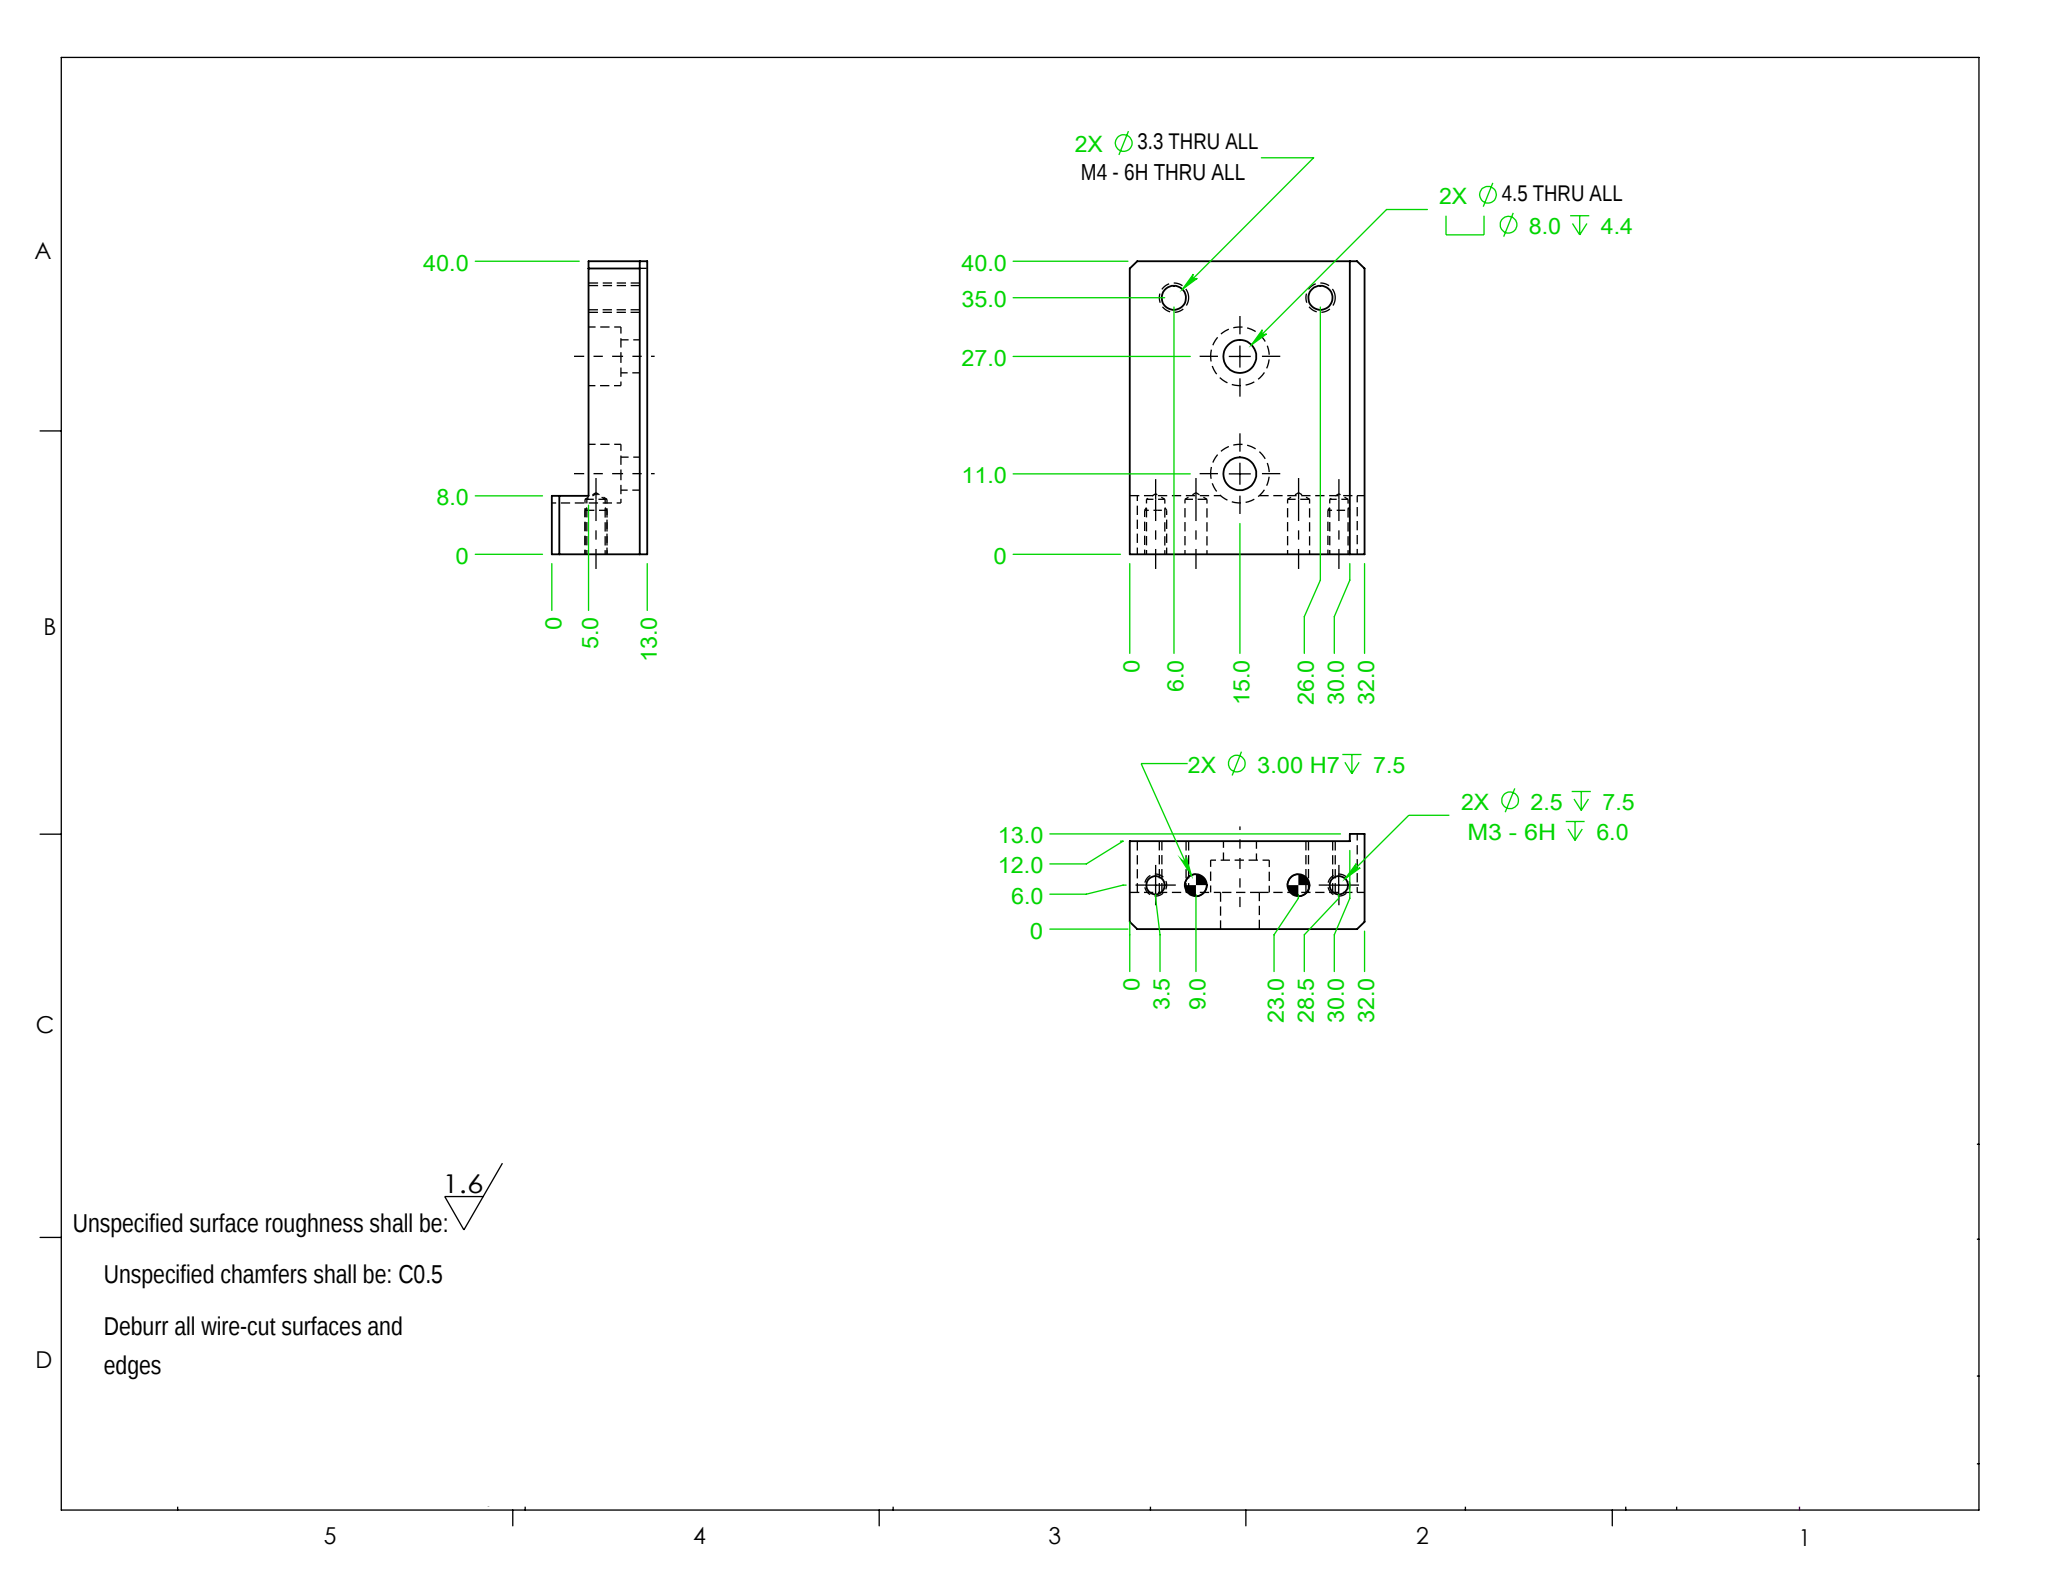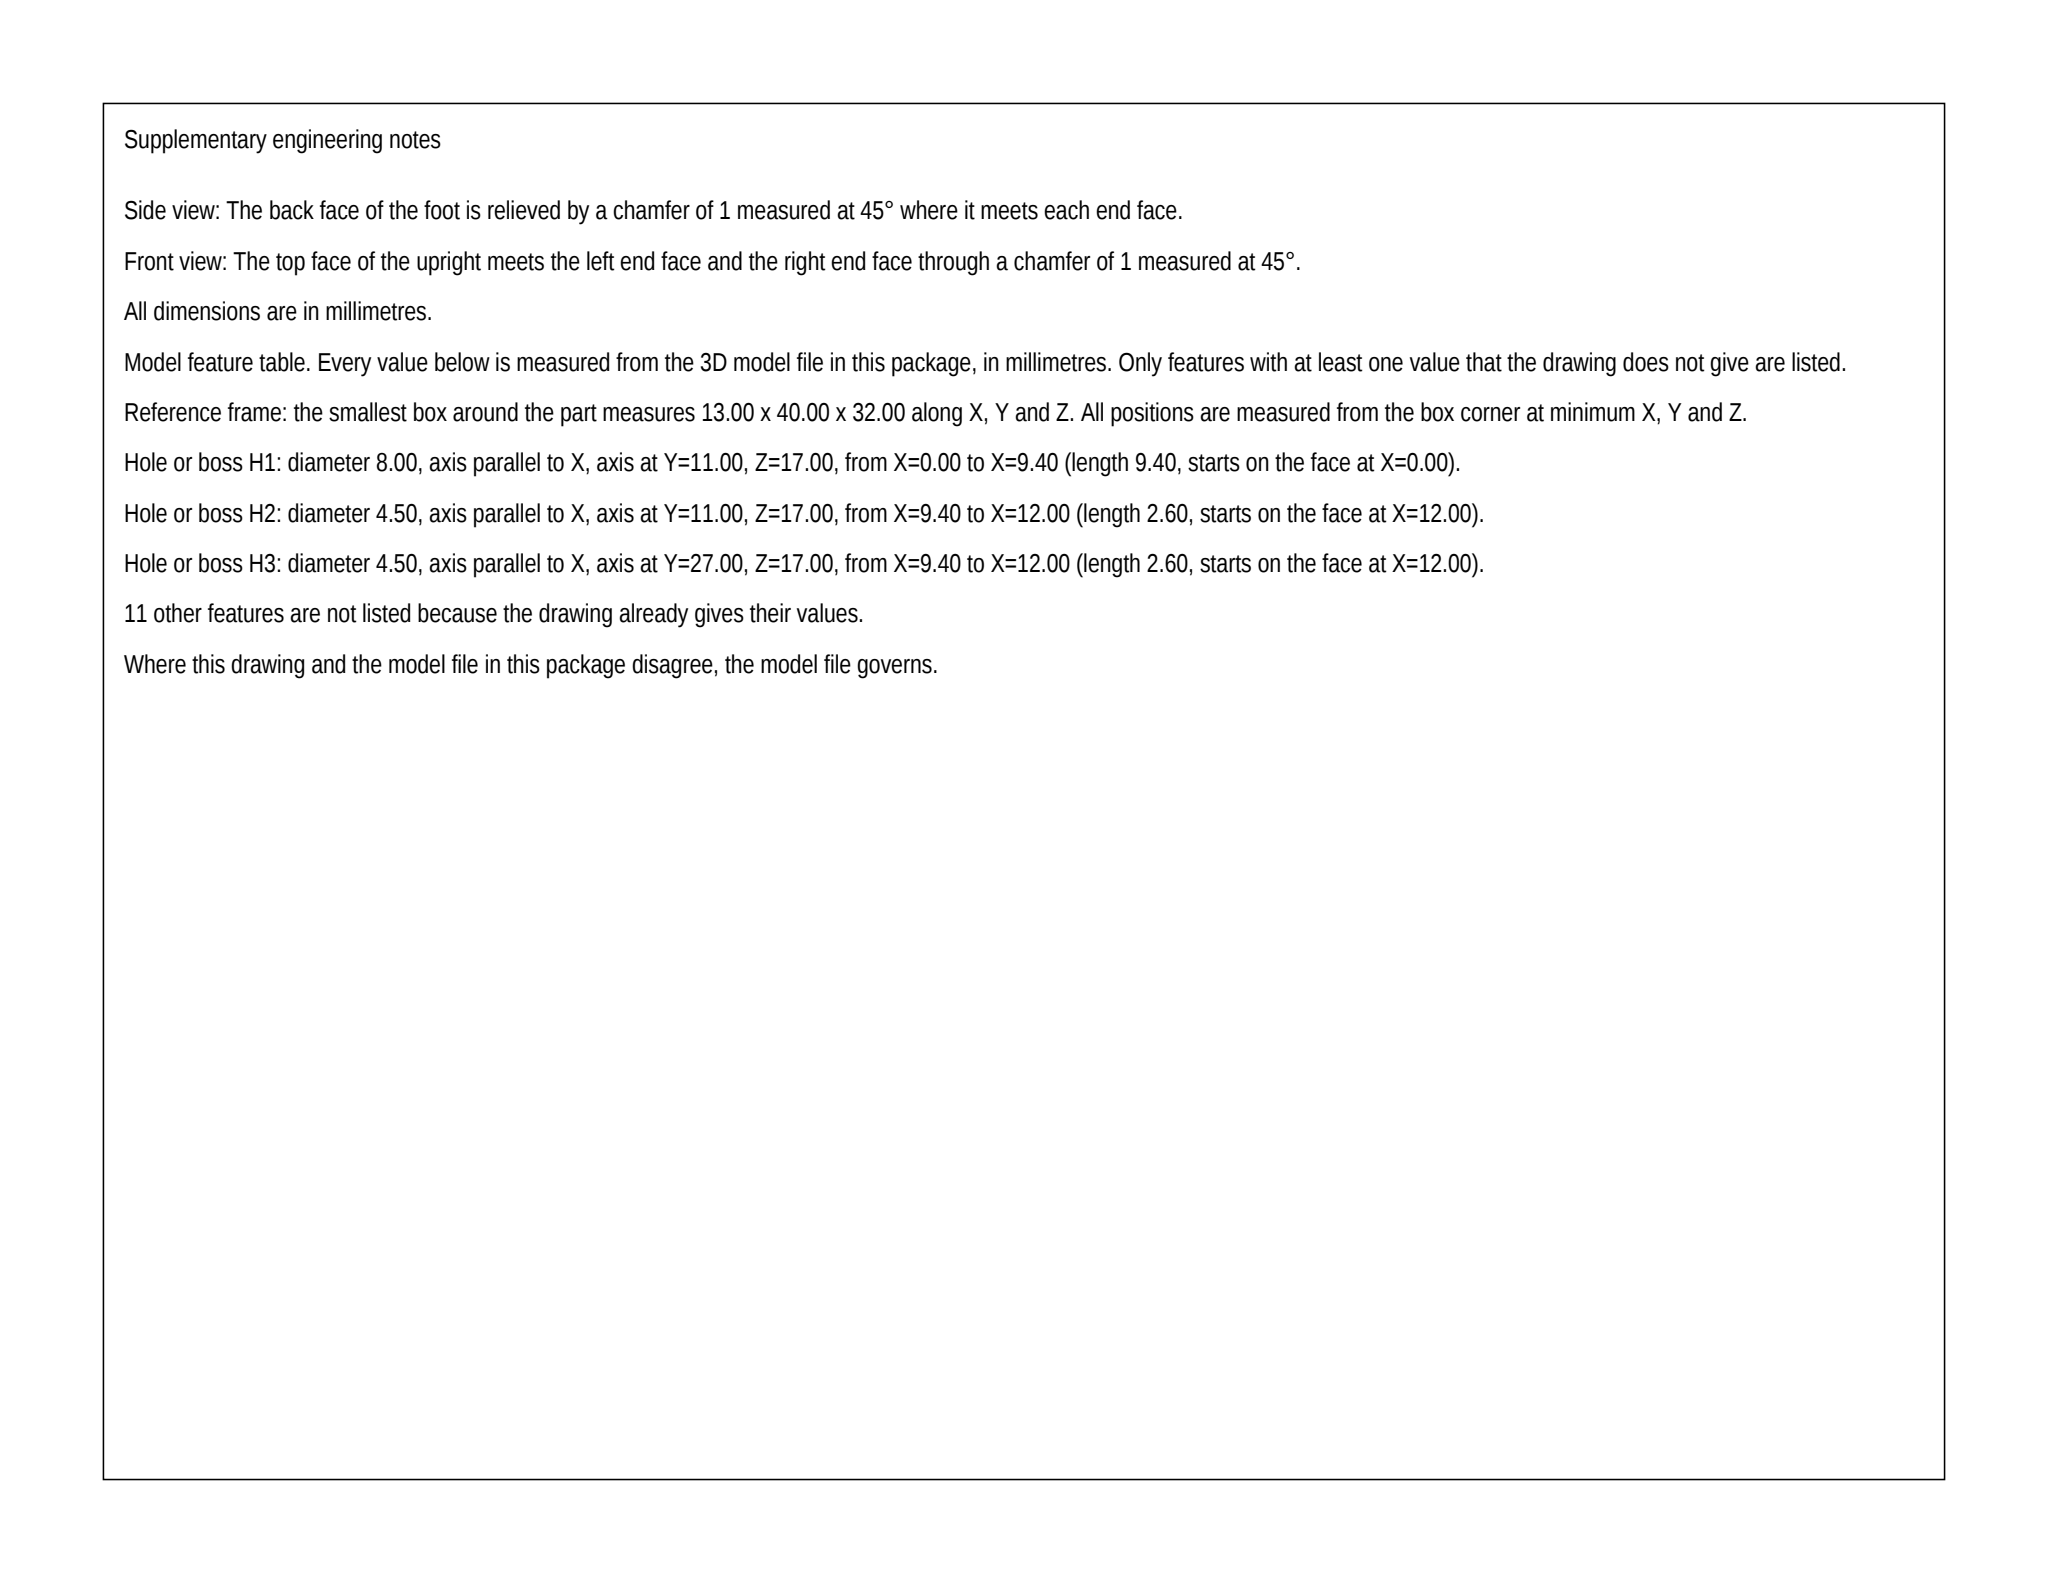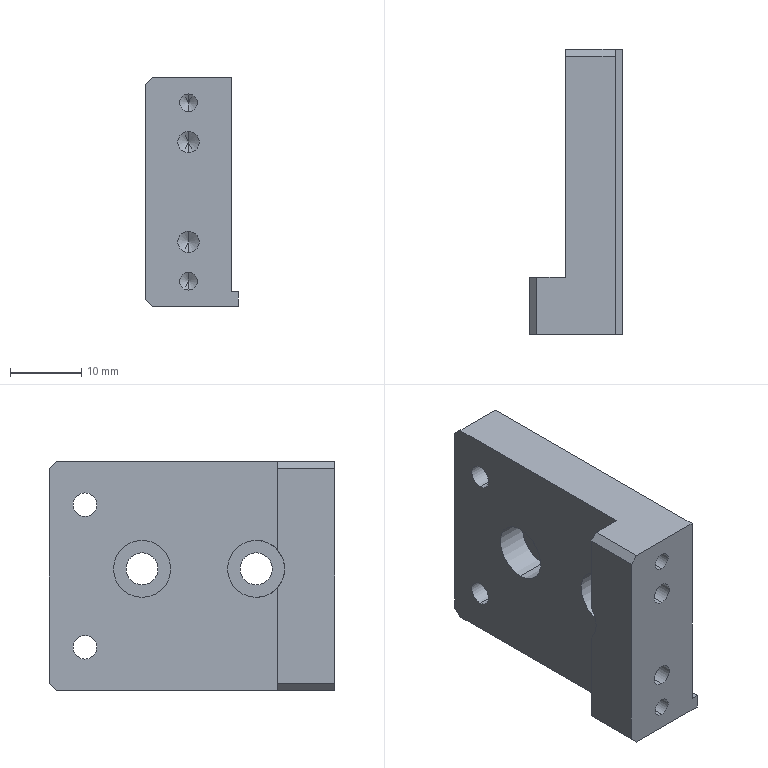Part | SolidWorks | mm | 1 solid | 45 faces | box 13 x 40 x 32 mm | volume 9455 mm3 | cylinder 20 | plane 17 | cone 8 | commonest cylinder face diameters 3.3 x4 8 x4 4.5 x4 3 x4 2.5 x4
build123d program:
from build123d import *

# Parameters (mm, degrees)
EXTRUDE_THIN1_DEPTH                            = 32
SKETCH2_W                                      = 30
SKETCH2_H                                      = 40
CUT_EXTRUDE1_DEPTH                             = 1
M3_TAPPED_HOLE1_D                              = 2.5
M3_TAPPED_HOLE1_DEPTH                          = 7.5
M3_TAPPED_HOLE1_TIP                            = 0.7511
SIZE_MM_DOWEL_PIN_HOLE1_D                      = 3
SIZE_MM_DOWEL_PIN_HOLE1_DEPTH                  = 7.5
SIZE_MM_DOWEL_PIN_HOLE1_TIP                    = 0.9013
CHAMFER1_SIZE                                  = 1
M4_HEX_SOCKET_HEAD_CAP_SCREW_CBORE1_AT_2_COUNT = 2
M4_HEX_SOCKET_HEAD_CAP_SCREW_CBORE1_AT_2_PITCH = 16
SKETCH11_R                                     = 4
CUT_EXTRUDE2_DEPTH                             = 9.4
M4_TAPPED_HOLE1_D                              = 3.3


with BuildPart() as part:
    # Sketch1 → Extrude-Thin1 (new body)
    with BuildSketch(Plane.XY):
        Polygon((0, 40), (0, 0), (-13, 0), (-13, 8), (-8, 8), (-8, 40), align=None)
    extrude(amount=EXTRUDE_THIN1_DEPTH)

    # Sketch2 → Cut-Extrude1 (cut)
    with BuildSketch(Plane(origin=(0, 0, 0), x_dir=(0, 0, -1), z_dir=(1, 0, 0))):
        with Locations((-17, 20)):
            Rectangle(SKETCH2_W, SKETCH2_H)
    extrude(amount=-CUT_EXTRUDE1_DEPTH, mode=Mode.SUBTRACT)

    # M3 Tapped Hole1
    with Locations(Plane(origin=(0, 0, 0), x_dir=(-1, 0, 0), z_dir=(0, -1, 0))):
        with Locations((7, -3.5), (7, -28.5)):
            Hole(M3_TAPPED_HOLE1_D / 2, depth=M3_TAPPED_HOLE1_DEPTH)
            with Locations((0, 0, -(M3_TAPPED_HOLE1_DEPTH + M3_TAPPED_HOLE1_TIP / 2))):  # 118° drill point
                Cone(0, M3_TAPPED_HOLE1_D / 2, M3_TAPPED_HOLE1_TIP, mode=Mode.SUBTRACT)

    # Size mm Dowel Pin Hole1
    with Locations(Plane(origin=(0, 0, 0), x_dir=(-1, 0, 0), z_dir=(0, -1, 0))):
        with Locations((7, -9), (7, -23)):
            Hole(SIZE_MM_DOWEL_PIN_HOLE1_D / 2, depth=SIZE_MM_DOWEL_PIN_HOLE1_DEPTH)
            with Locations((0, 0, -(SIZE_MM_DOWEL_PIN_HOLE1_DEPTH + SIZE_MM_DOWEL_PIN_HOLE1_TIP / 2))):  # 118° drill point
                Cone(0, SIZE_MM_DOWEL_PIN_HOLE1_D / 2, SIZE_MM_DOWEL_PIN_HOLE1_TIP, mode=Mode.SUBTRACT)

    # Chamfer1
    chamfer1_edges = [part.edges().sort_by_distance(p)[0] for p in [
        (-4.5, 40, 32),
        (-4, 40, 0),
        (-13, 4, 0),
        (-13, 4, 32),
    ]]
    chamfer(chamfer1_edges, length=CHAMFER1_SIZE)

    # Sketch9 → M4 Hex Socket Head Cap Screw CBORE1 (revolve, cut)
    with BuildSketch(Plane(origin=(-8, 27, 17), x_dir=(0, 0, 1), z_dir=(0, 1, 0))):
        Polygon((0, 0), (0, 8), (2.25, 8), (2.25, 4.4), (4, 4.4), (4, 0), align=None)
    m4_hex_socket_head_cap_screw_cbore1 = revolve(axis=Axis((-14.35, 27, 17), (1, 0, 0)), mode=Mode.SUBTRACT)

    # M4 Hex Socket Head Cap Screw CBORE1 at 2: M4 Hex Socket Head Cap Screw CBORE1 ×2
    with Locations(*[(0, -i * M4_HEX_SOCKET_HEAD_CAP_SCREW_CBORE1_AT_2_PITCH, 0) for i in range(1, M4_HEX_SOCKET_HEAD_CAP_SCREW_CBORE1_AT_2_COUNT)]):
        add(m4_hex_socket_head_cap_screw_cbore1, mode=Mode.SUBTRACT)

    # Sketch11 → Cut-Extrude2 (cut)
    with BuildSketch(Plane.ZY.offset(13)):
        with Locations((17, 11)):
            Circle(SKETCH11_R)
    extrude(amount=-CUT_EXTRUDE2_DEPTH, mode=Mode.SUBTRACT)

    # M4 Tapped Hole1 (through all)
    with Locations(Plane.ZY.offset(8)):
        with Locations((6, 35), (26, 35)):
            Hole(M4_TAPPED_HOLE1_D / 2)


solid = part.part